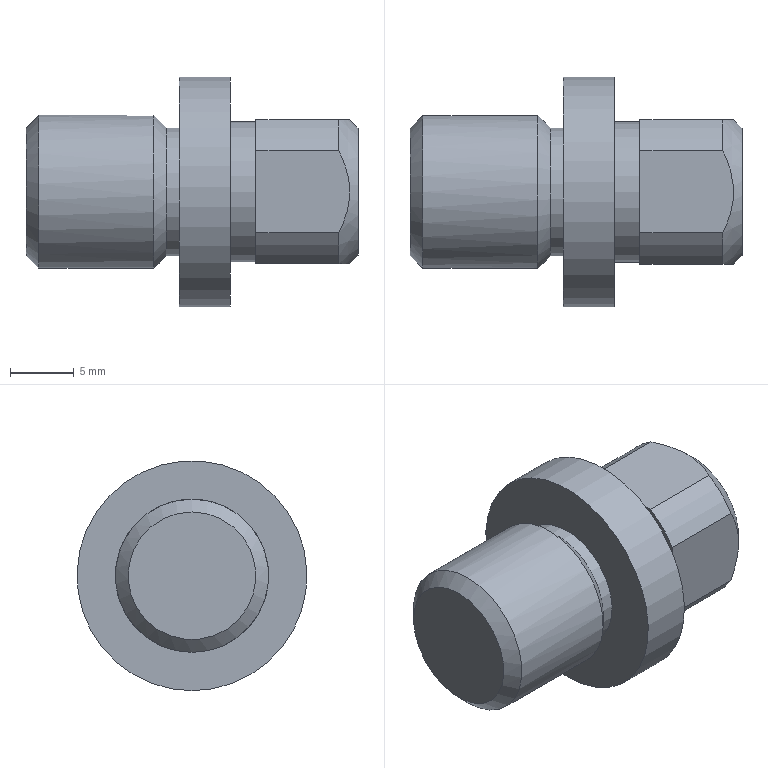Component | NX | LOC_SCREW | 1 solid | 20 faces | volume 3413 mm3 | plane 9 | cylinder 8 | cone 3 | commonest cylinder face diameters 13 x4 12 x1 10 x1 18 x1 11 x1